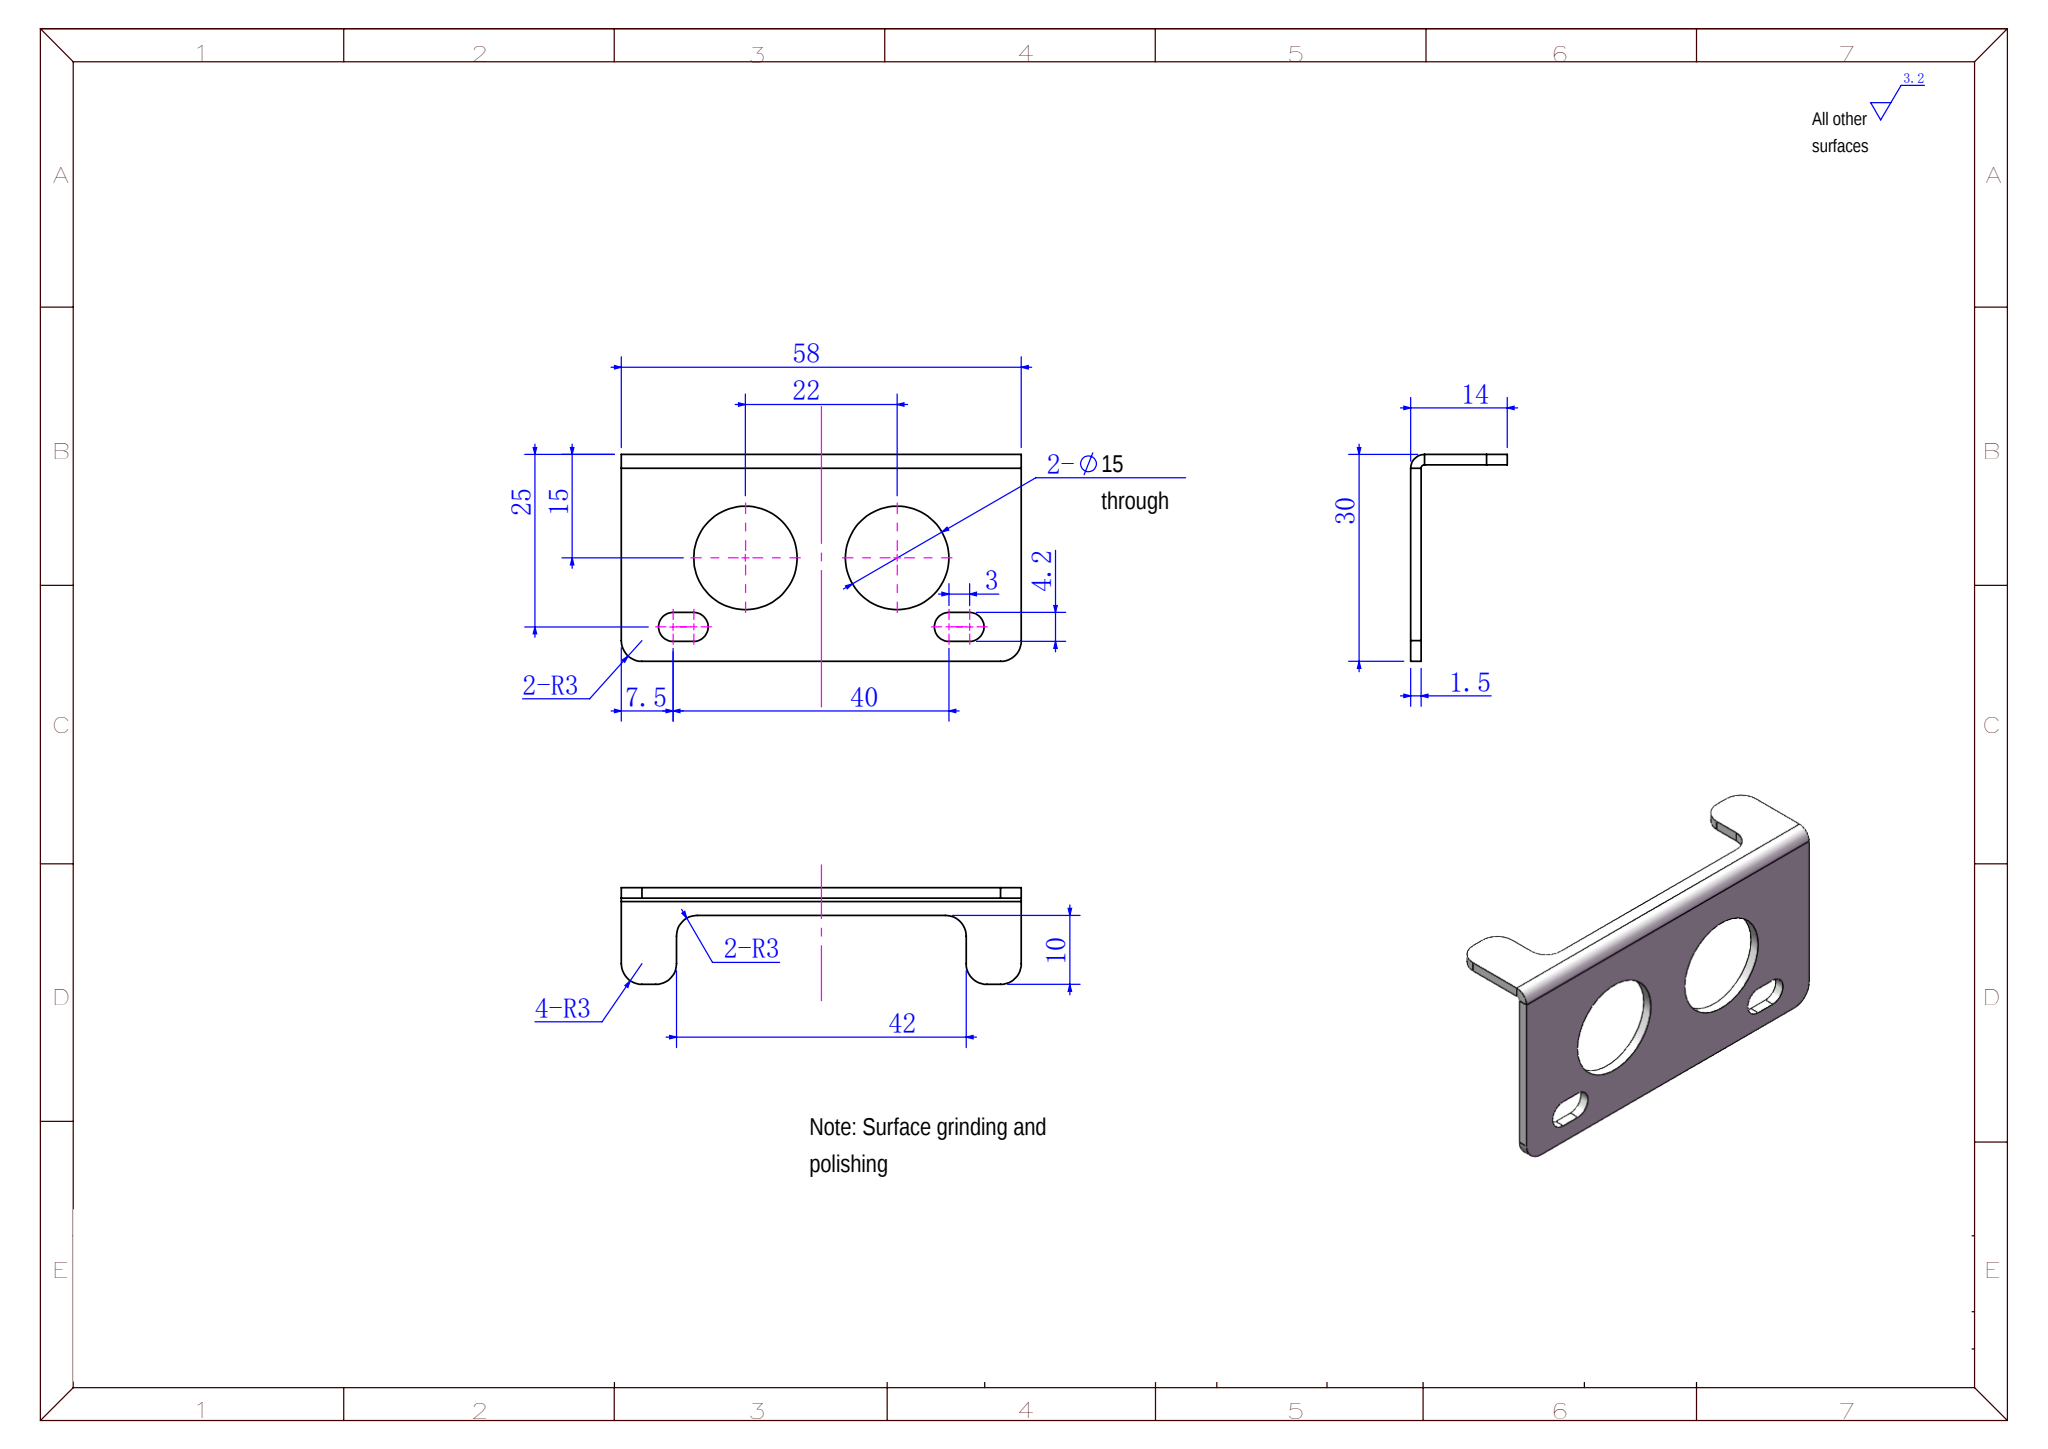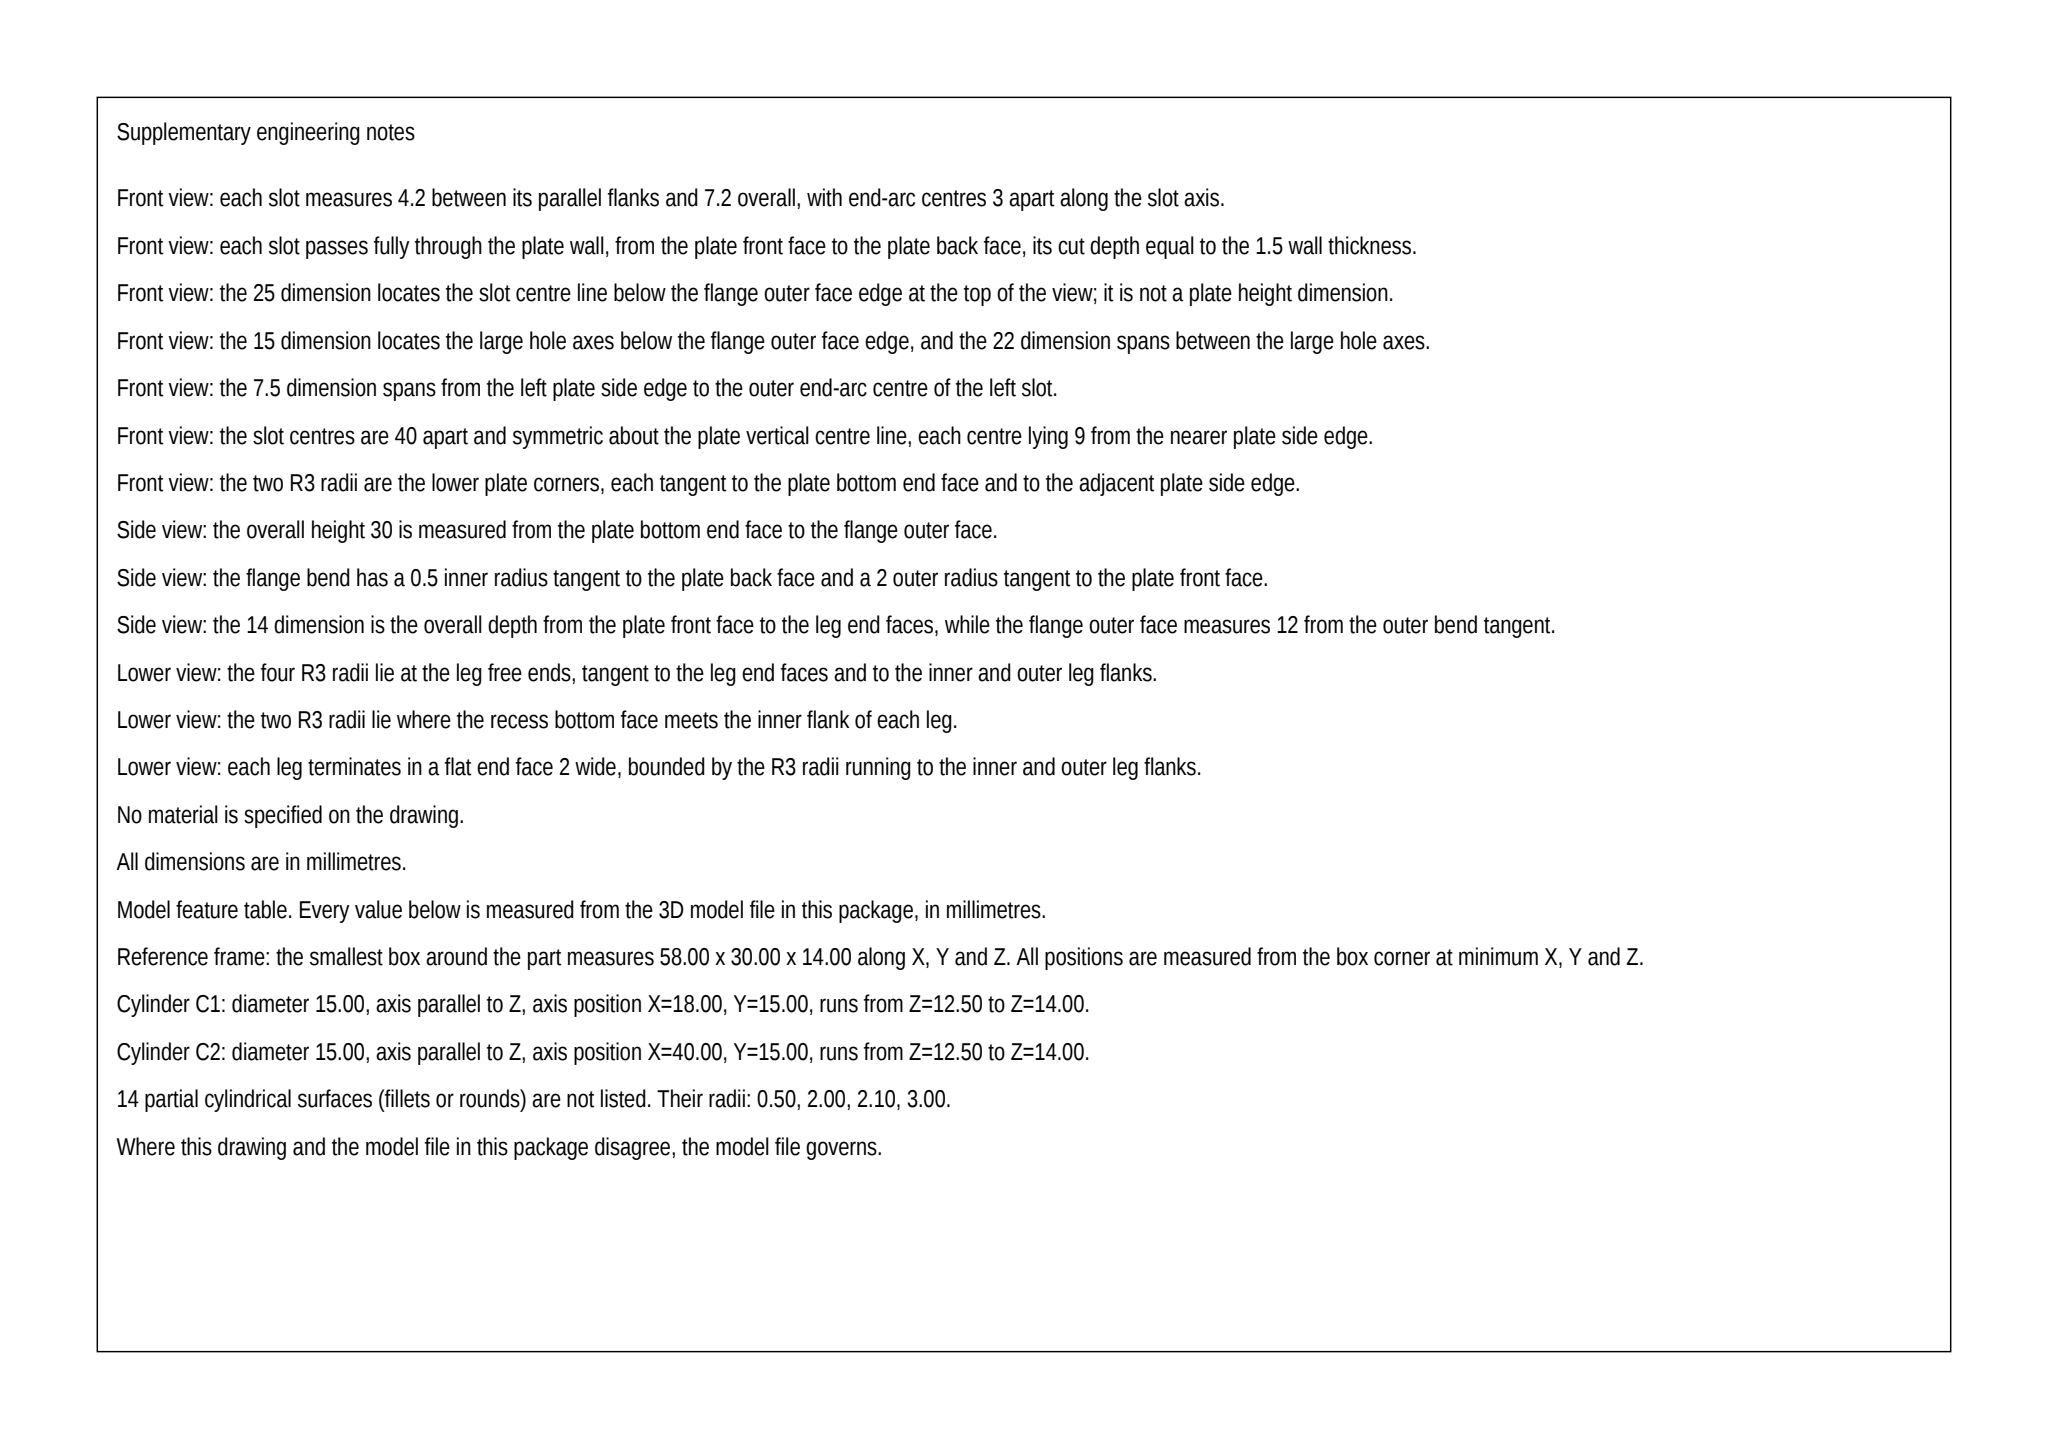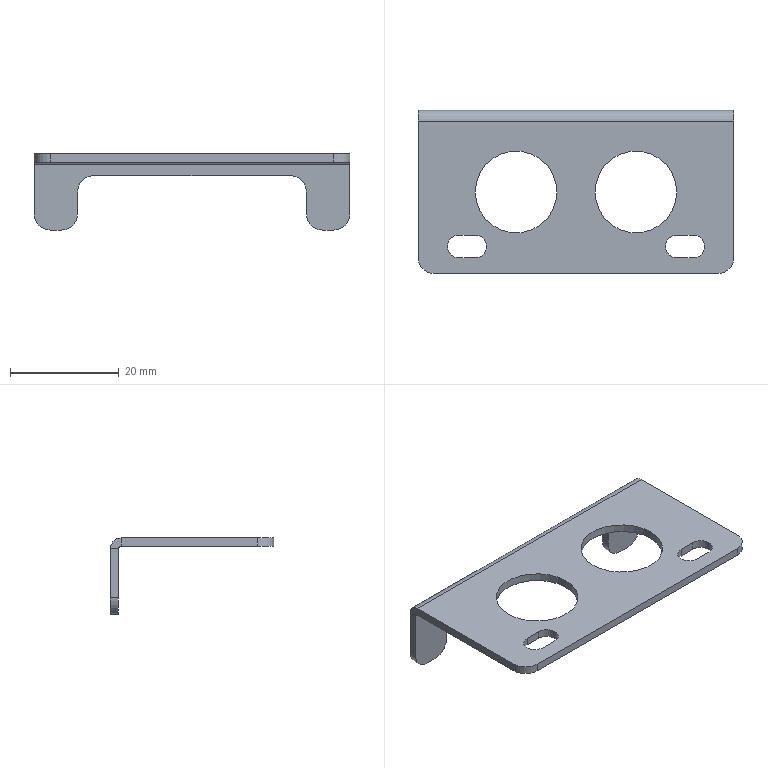Part | SolidWorks | mm | 1 solid | 40 faces | box 58 x 30 x 14 mm | volume 2400 mm3 | cylinder 20 | plane 20 | commonest cylinder face diameters 6 x8 4.2 x6 15 x4 4 x1 1 x1
Drawing notes:
BEND BETWEEN 30 PLATE & 14 FLANGE: R0.5 INSIDE, R2 OUTSIDE | from the solid: X-axis cyls dia 1.0 and dia 4.0, both at (y=28, z=12), len 58 = inner/outer bend radii at 1.5 thk 90 deg bend